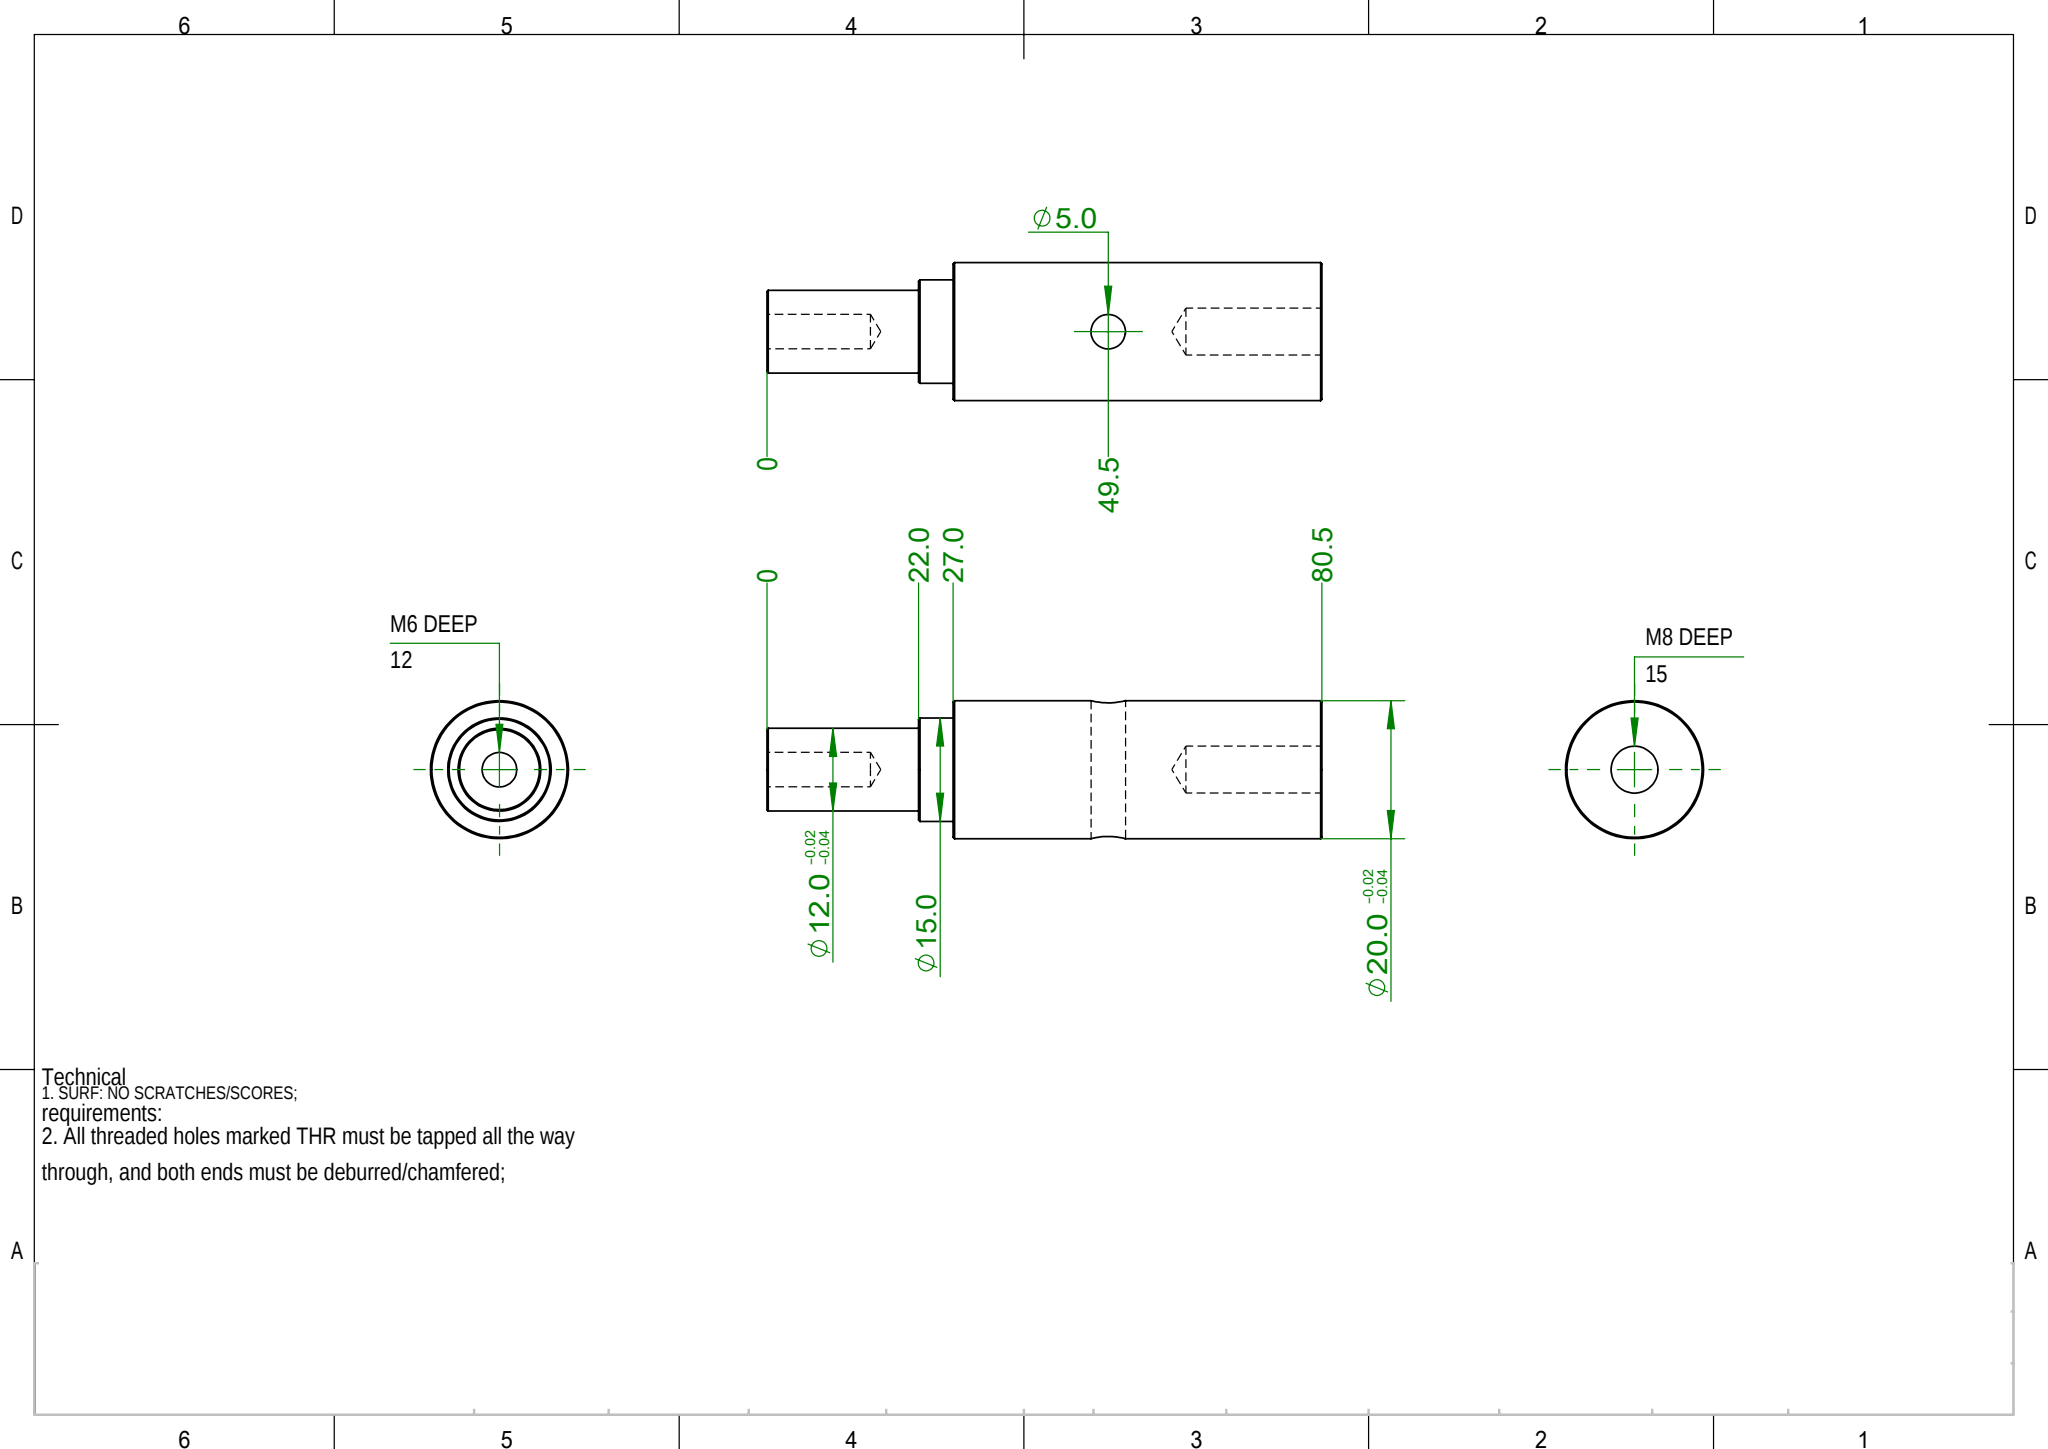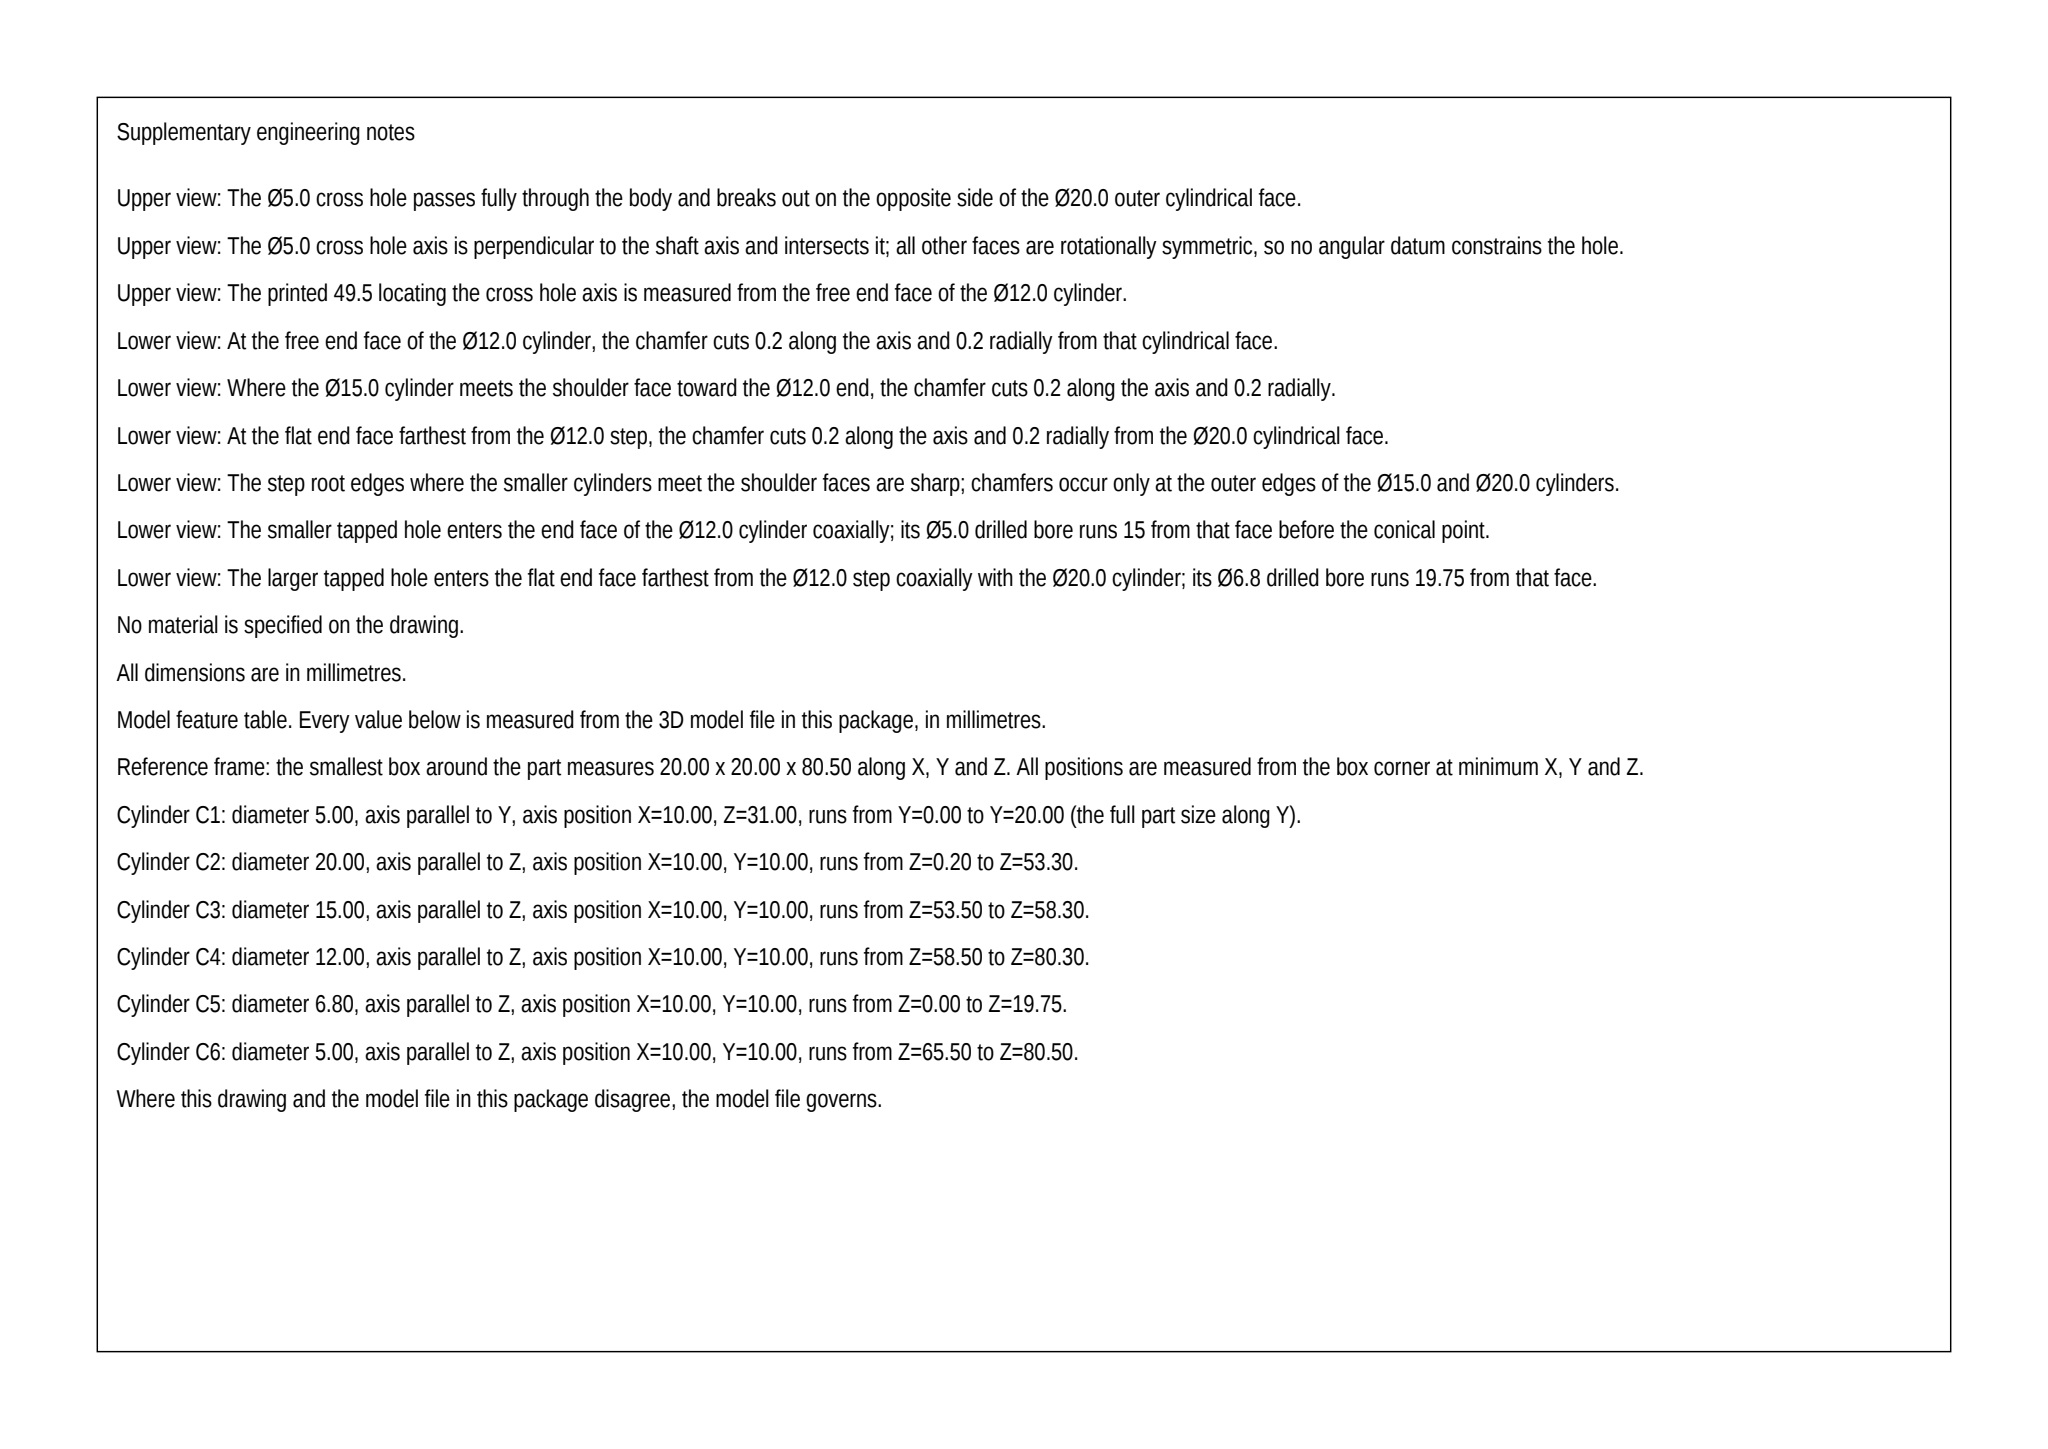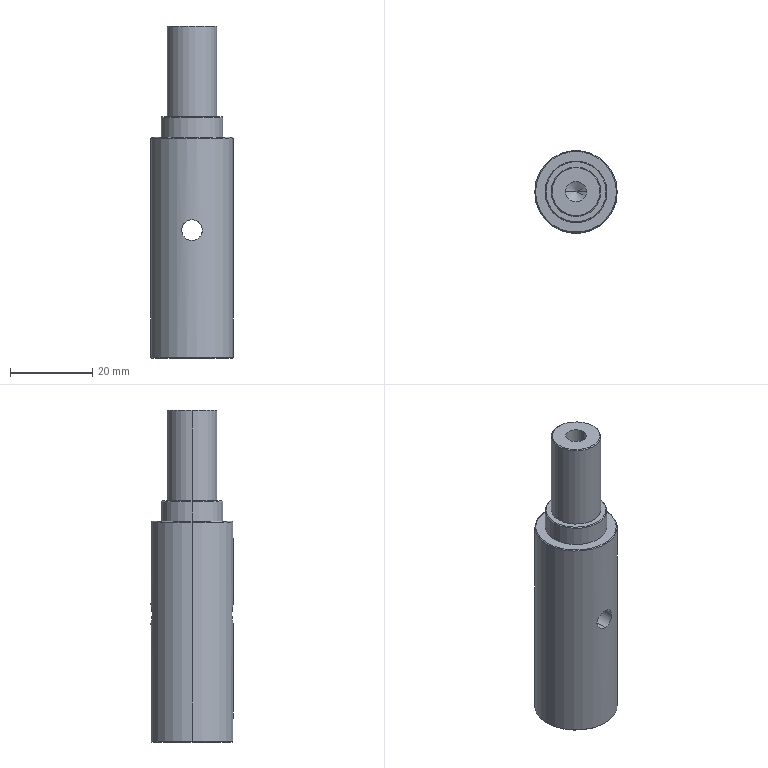Part | SolidWorks | mm | 1 solid | 28 faces | box 20 x 20 x 80.5 mm | volume 18739 mm3 | cylinder 12 | cone 12 | plane 4 | commonest cylinder face diameters 5 x4 6.8 x2 20 x2 12 x2 15 x2
Drawing notes:
UNSPECIFIED CHAMFERS C0.2 x 45 DEG | from the solid: 90 deg cones at ref Ø11.6, Ø14.6, Ø19.6, Ø20.0; 0.2 axial each (21.8+4.8+53.1+4x0.2=80.5)
M6 DP 12: TAP DRILL Ø5.0 DP 15, 118 DEG PT | from the solid: cylinder [5.0,z,(10,10),15] + cone 118 deg ref dia 5.0
M8 DP 15: TAP DRILL Ø6.8 DP 19.75, 118 DEG PT | from the solid: cylinder [6.8,z,(10,10),19.75] + cone 118 deg ref dia 6.8
ALL DIMS IN MM | from the solid: STEP model units mm; bbox 20.0 x 20.0 x 80.5